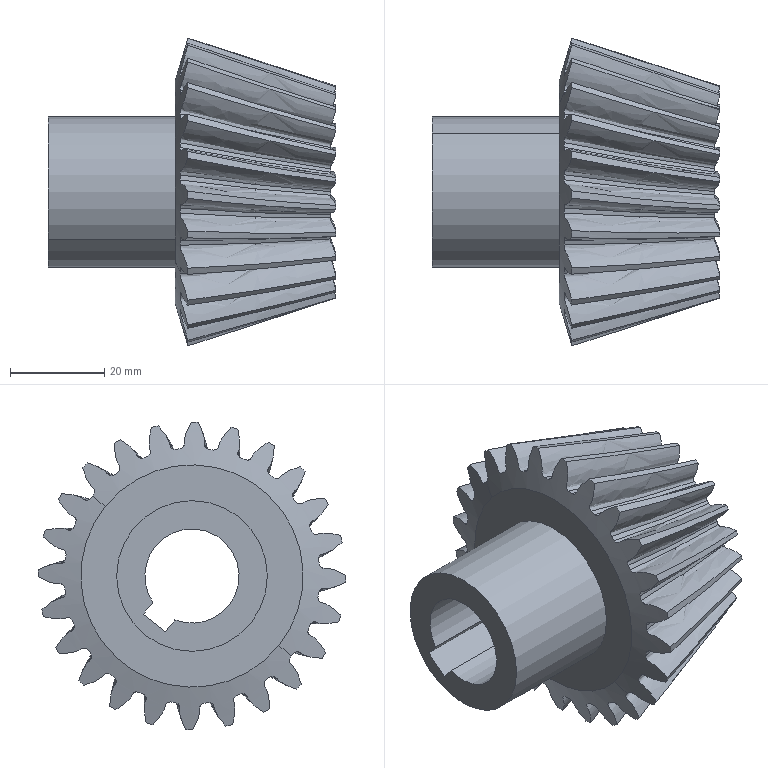Component | SolidWorks | BevelGear24_2.5-1 | 1 solid | 135 faces | volume 69320 mm3 | spline 72 | cone 52 | plane 6 | cylinder 5 | commonest cylinder face diameters 20 x3 32 x2